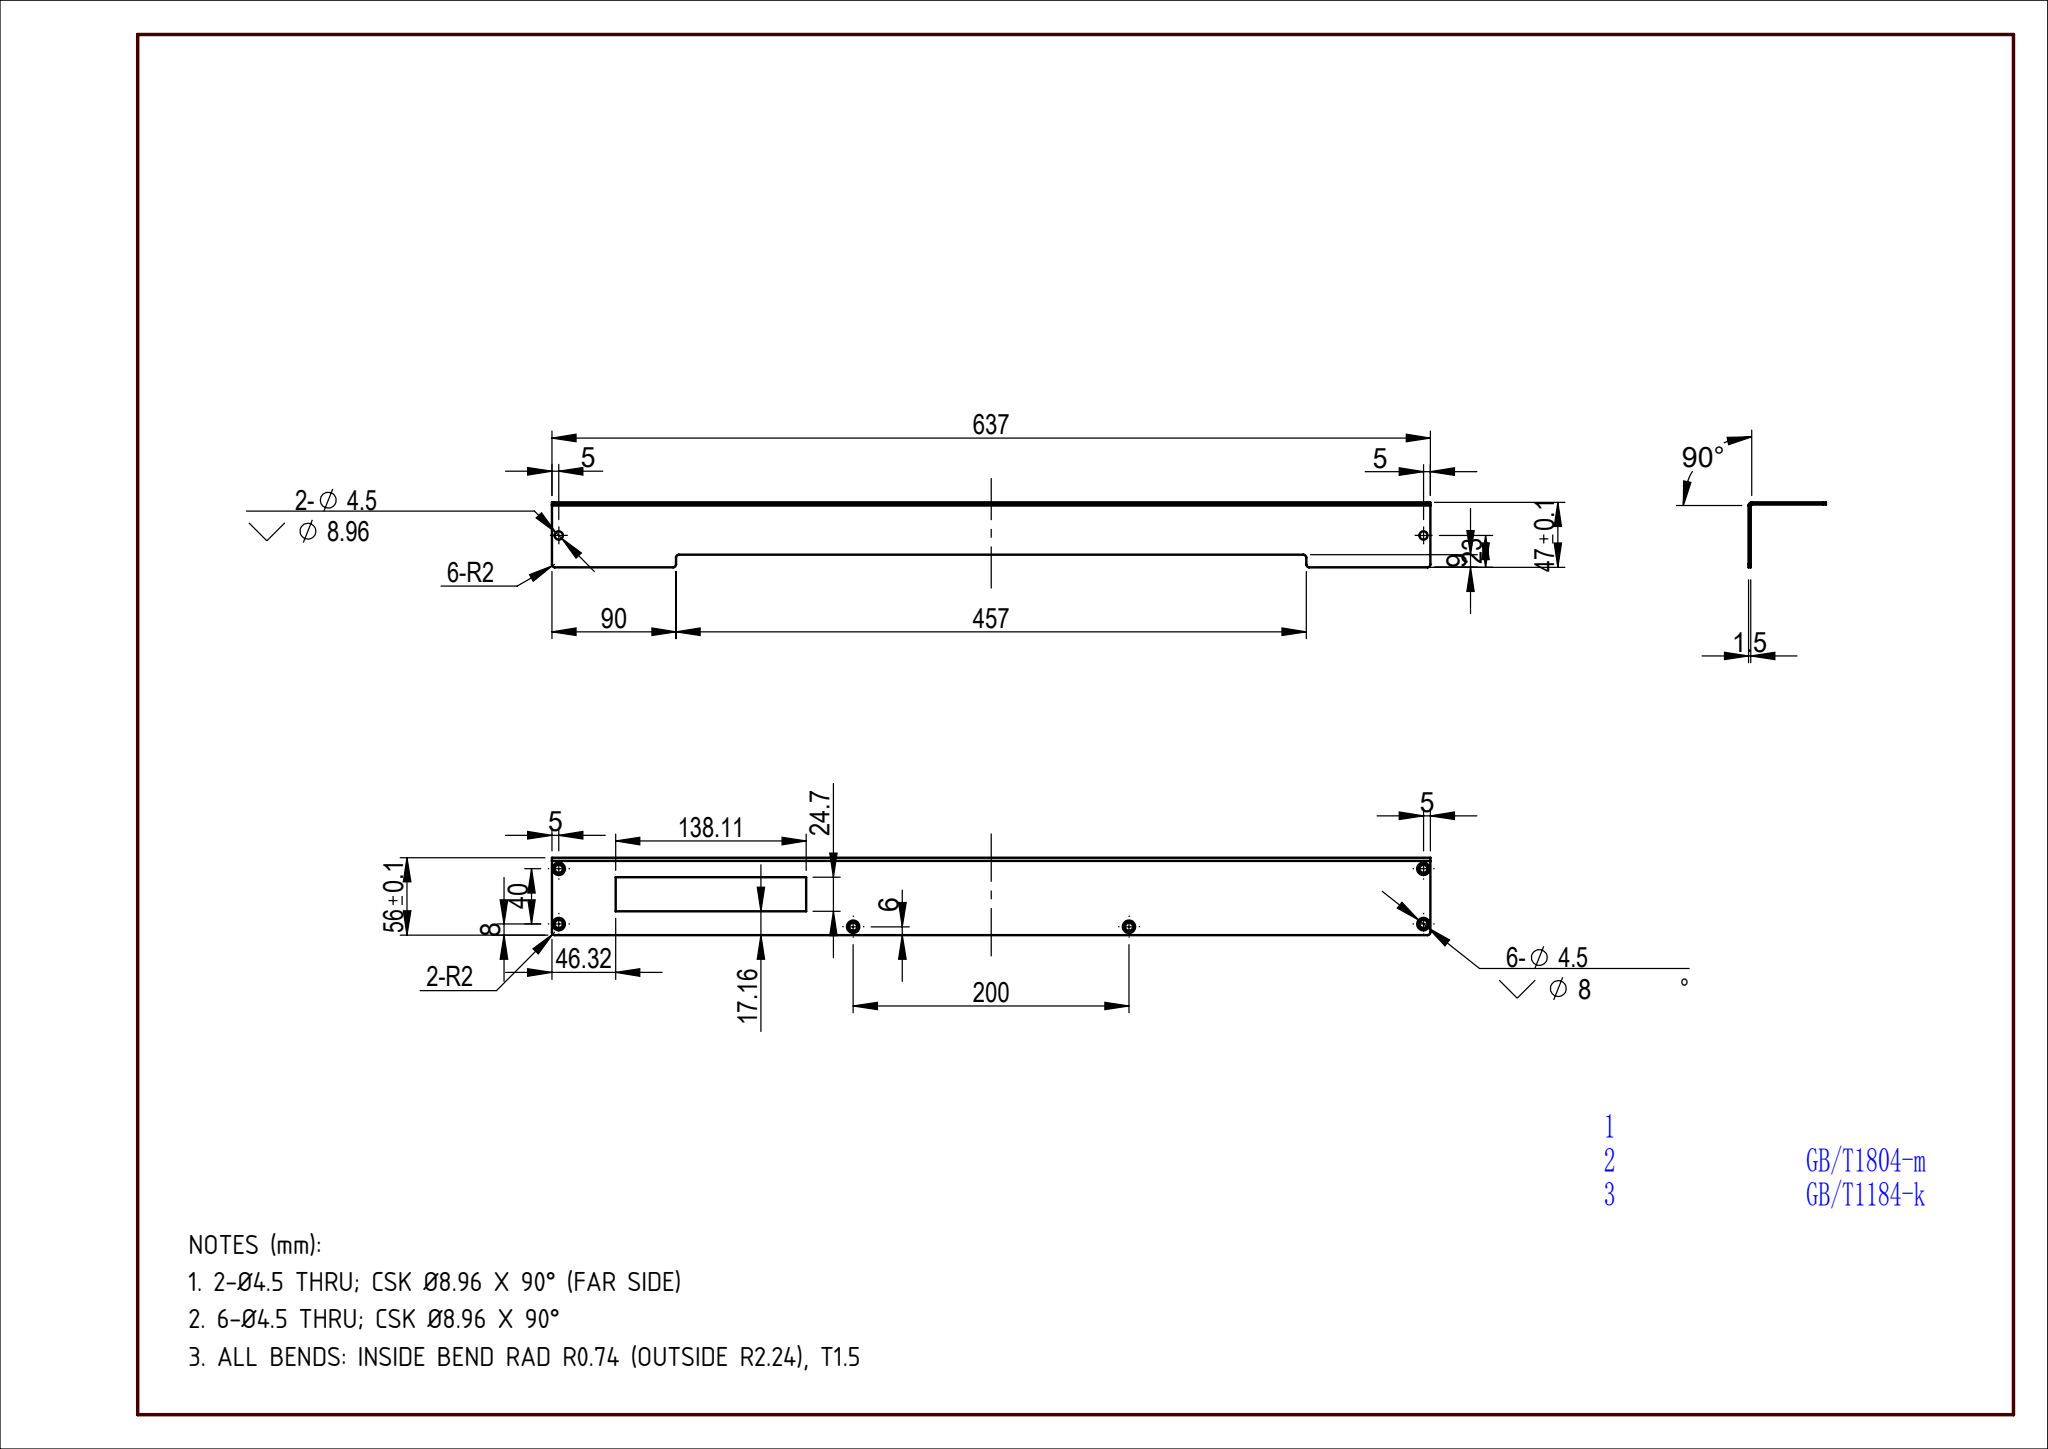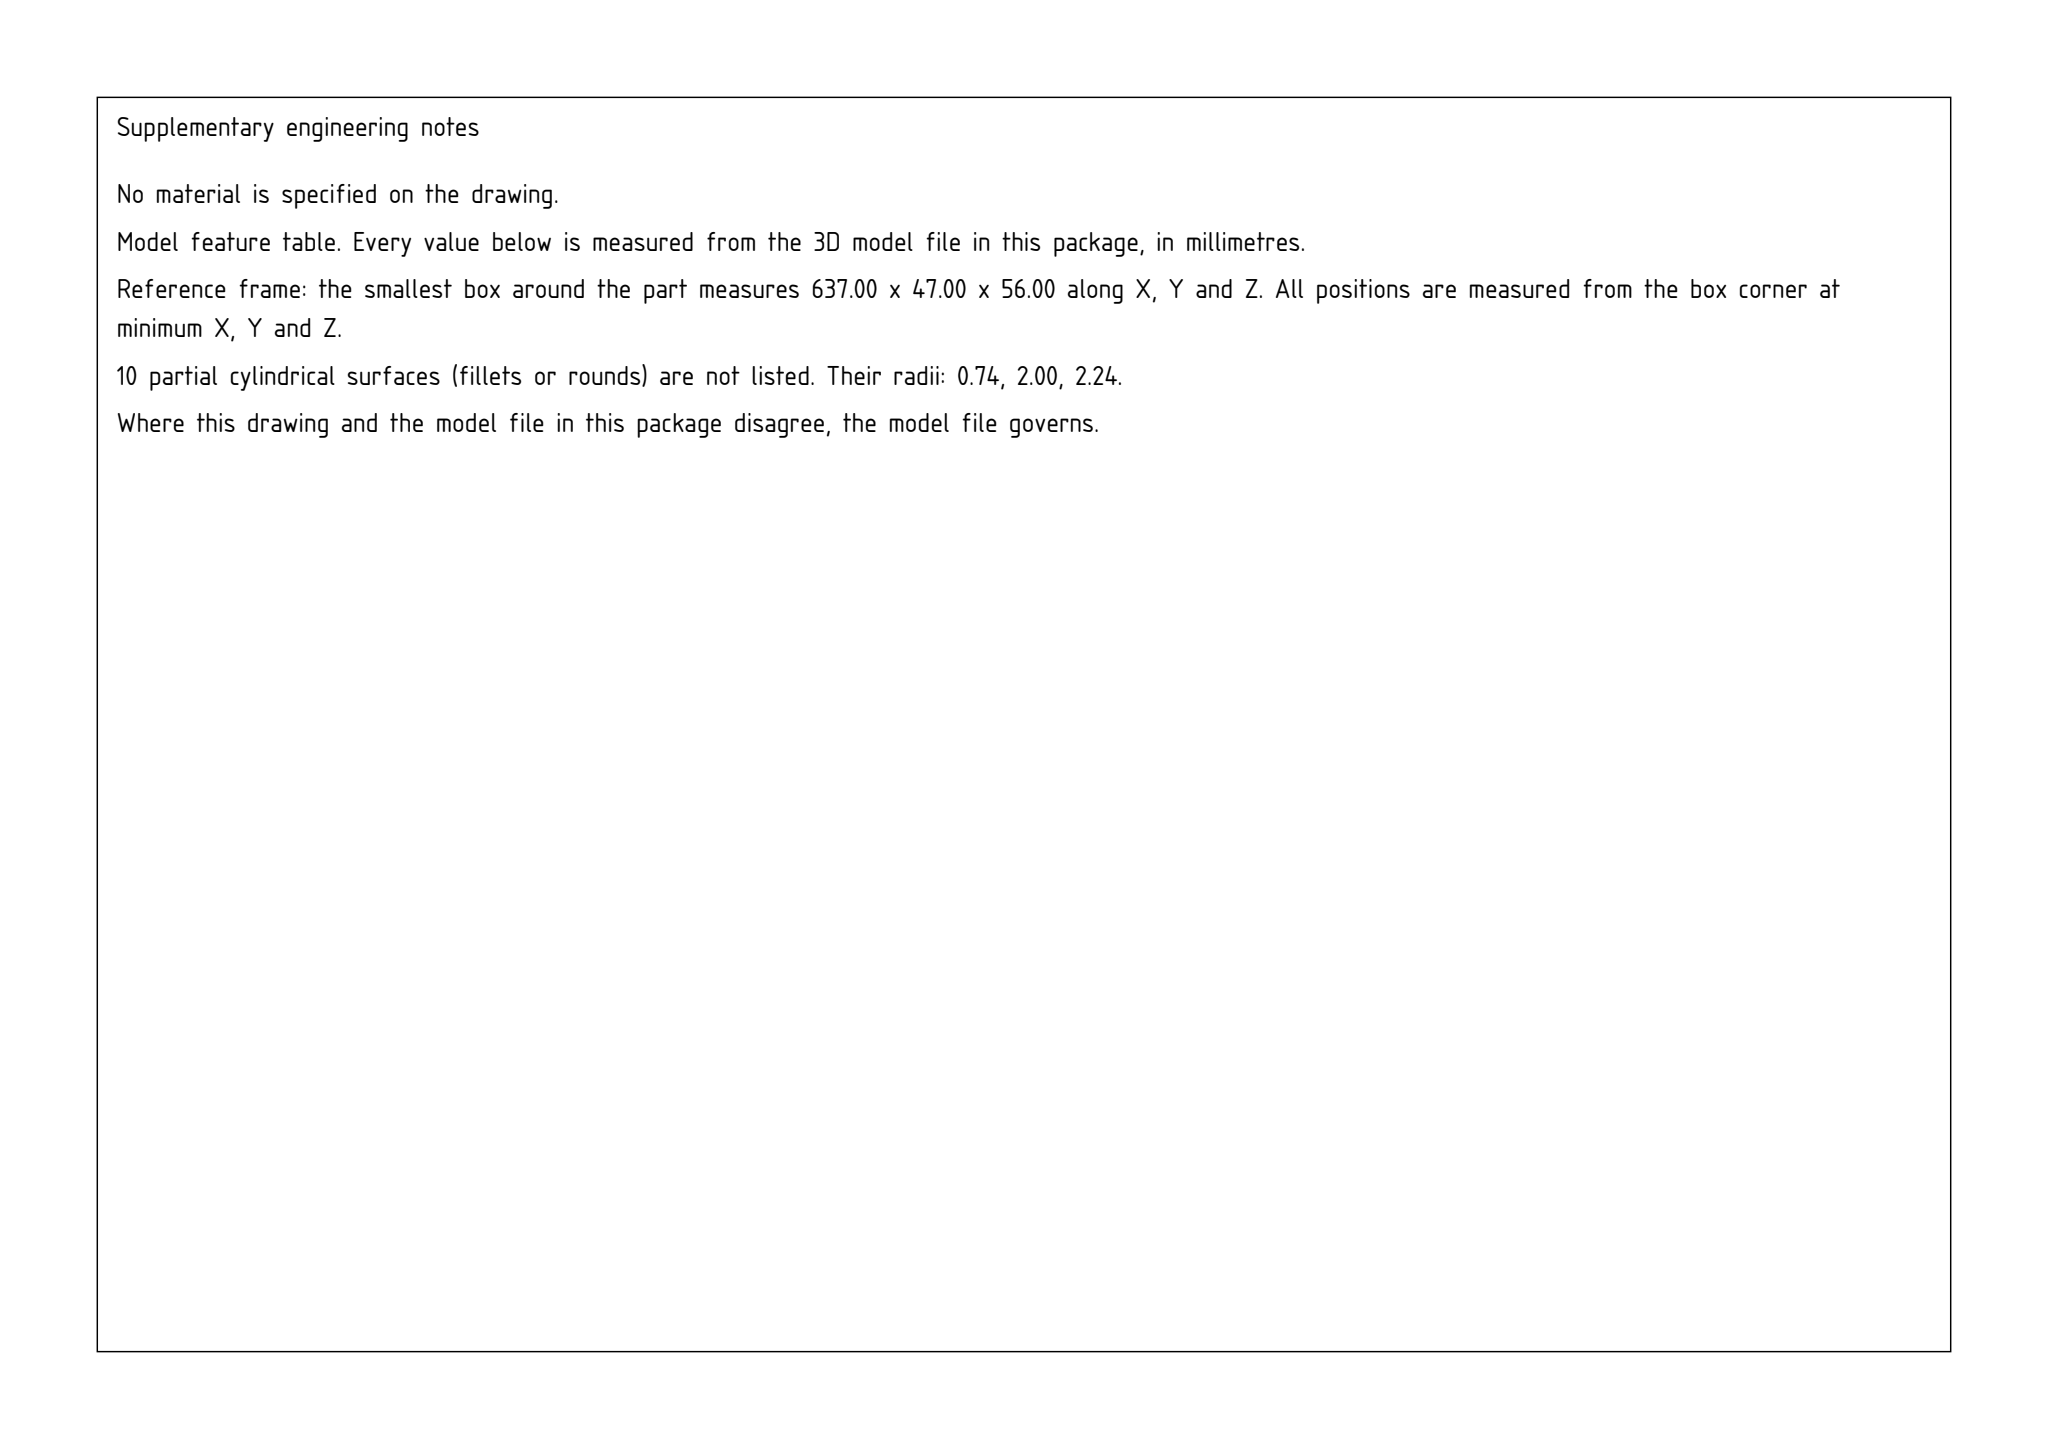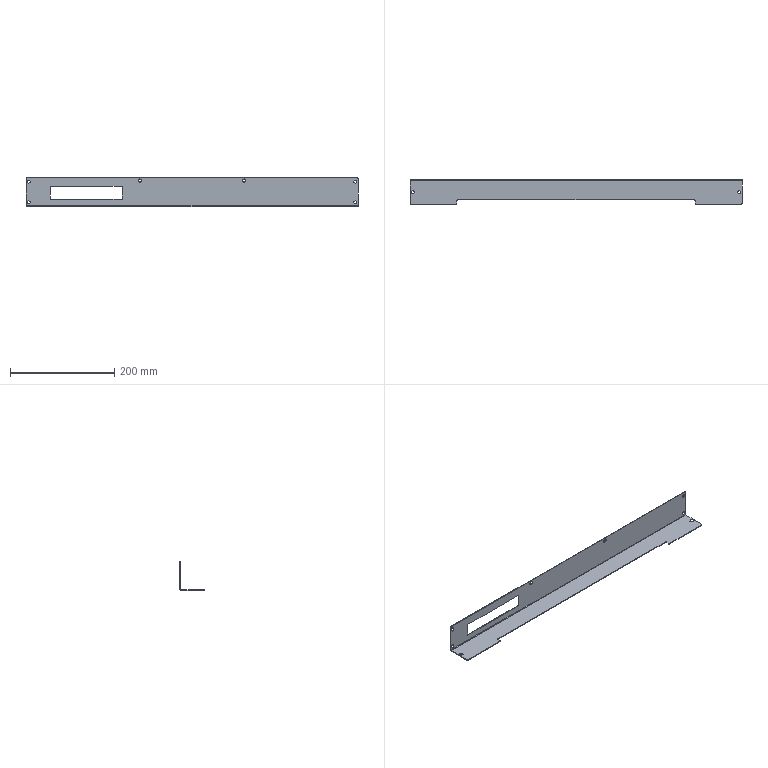Part | SolidWorks | mm | 1 solid | 46 faces | box 637 x 47 x 56 mm | volume 84551 mm3 | plane 20 | cone 16 | cylinder 10 | commonest cylinder face diameters 4 x8 4.473 x1 1.473 x1
Drawing notes:
2-Ø4.5 THRU; CSK Ø8.96 X 90° (FAR SIDE) | from the solid: cones[included_angle,ref_dia] = [[90.0, 8.96, 16]]; Ø4.0 holes thru 1.5 wall at x=2,635 (y-axis)
6-Ø4.5 THRU; CSK Ø8.96 X 90° | from the solid: cones[included_angle,ref_dia] = [[90.0, 8.96, 16]]; six Ø4.0 z-axis holes at x=2,88,92,545,549,635
ALL BENDS: INSIDE BEND RAD R0.74 (OUTSIDE R2.24), T1.5 | from the solid: cylinders dia 1.473 and 4.473, axis x, pos y44.76 z2.24, length 637; wall thk 1.5 (z 0-1.5)